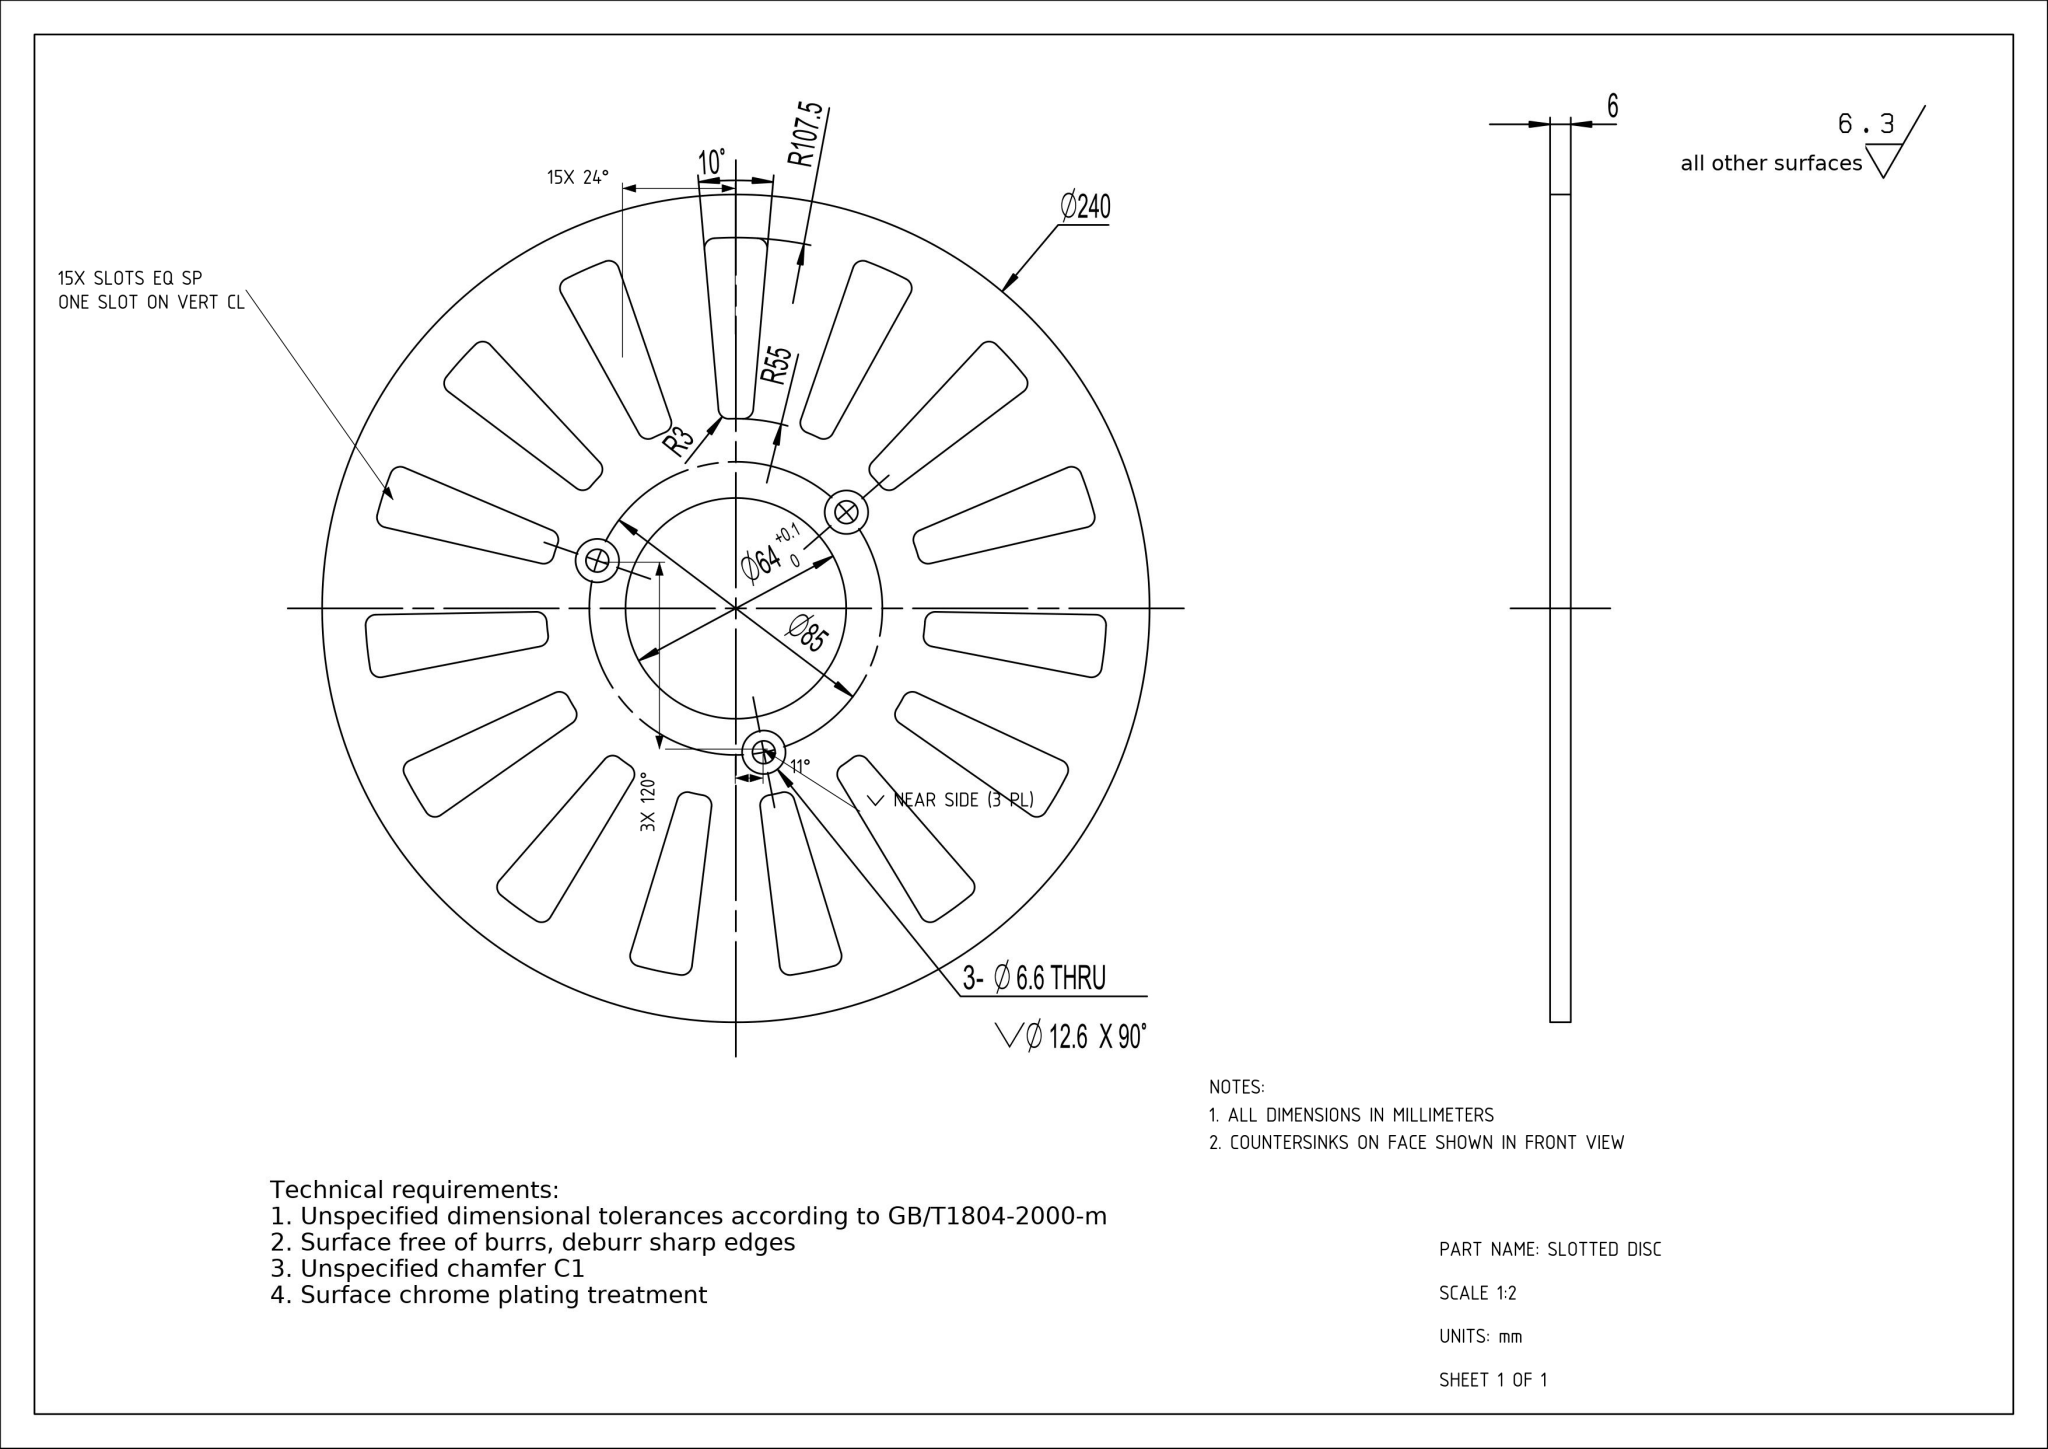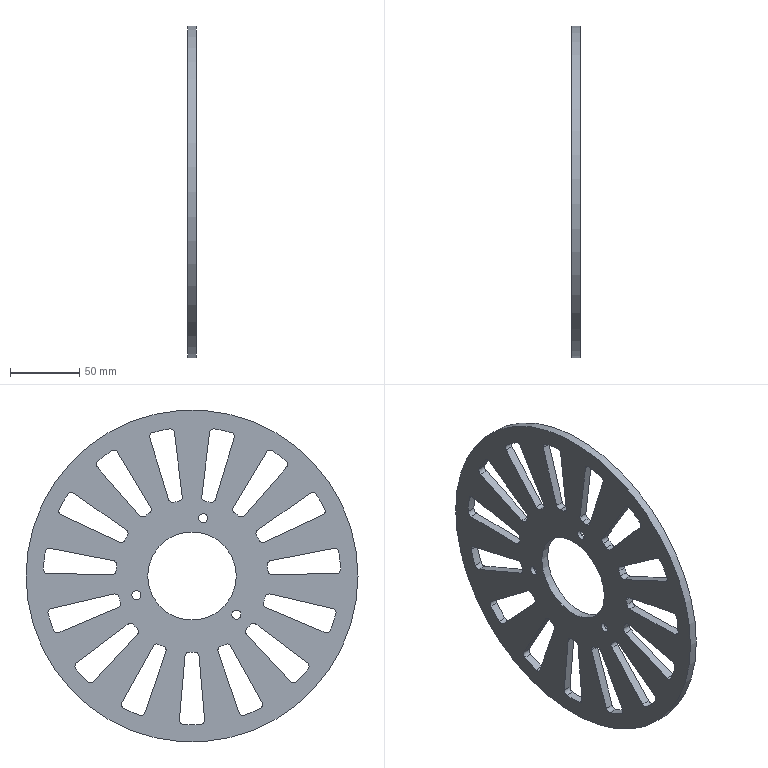Part | NX | mm | 1 solid | 130 faces | box 6 x 240 x 240 mm | volume 184831 mm3 | cylinder 95 | plane 32 | cone 3 | commonest cylinder face diameters 6 x60 215 x15 110 x15 6.6 x3 240 x1 64 x1